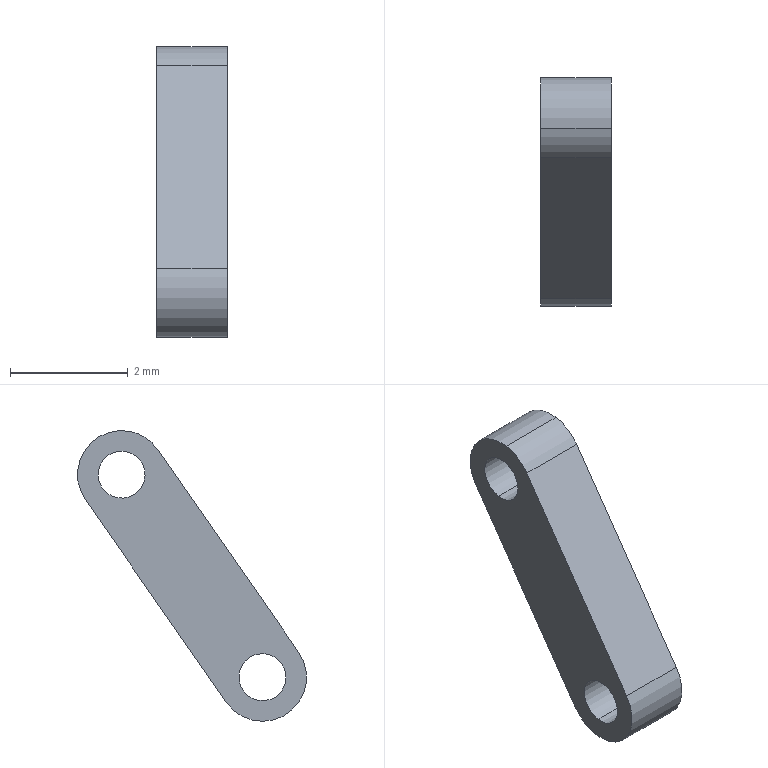Component | SolidWorks | RearWingYoke-4 | 1 solid | 11 faces | box 1.2 x 3.9 x 4.95 mm | volume 8 mm3 | cylinder 7 | plane 4 | commonest cylinder face diameters 0.8 x4 1.5 x3
build123d program:
from build123d import *

# Parameters (mm, degrees)
SKETCH1_R           = 0.4
BOSS_EXTRUDE1_DEPTH = 1.2


with BuildPart() as part:
    # Sketch1 → Boss-Extrude1 (new body)
    with BuildSketch(Plane.XY):
        with BuildLine():
            Line((-4.52, 1.96), (-7.547, 4.871))
            ThreePointArc((-7.547, 4.871), (-7.567, 5.932), (-6.507, 5.952))
            Line((-6.507, 5.952), (-3.48, 3.04))
            ThreePointArc((-3.48, 3.04), (-3.46, 1.98), (-4.52, 1.96))
        make_face()
        with Locations((-4, 2.5)):
            Circle(SKETCH1_R, mode=Mode.SUBTRACT)
        with Locations((-7.027, 5.412)):
            Circle(SKETCH1_R, mode=Mode.SUBTRACT)
    extrude(amount=BOSS_EXTRUDE1_DEPTH)


solid = part.part

# Placed as in the assembly
solid = solid.moved(Location((18.1, 10.831, 11.183), (-78.711, -90, 0)))
STEP:
#1=COLOUR_RGB('',0.7922,0.8196,0.9333);
#2=FILL_AREA_STYLE_COLOUR('',#1);
#3=FILL_AREA_STYLE('',(#2));
#4=SURFACE_STYLE_FILL_AREA(#3);
#5=SURFACE_SIDE_STYLE('',(#4));
#6=SURFACE_STYLE_USAGE(.BOTH.,#5);
#7=PRESENTATION_STYLE_ASSIGNMENT((#6));
#8=CARTESIAN_POINT('',(0.7126,0.2888,0.3285));
#9=VERTEX_POINT('',#8);
#10=CARTESIAN_POINT('',(0.7126,0.2938,0.2974));
#11=VERTEX_POINT('',#10);
#12=CARTESIAN_POINT('',(0.7126,0.2913,0.3129));
#13=DIRECTION('',(1.,0.,0.));
#14=DIRECTION('',(0.,0.1577,-0.9875));
#15=AXIS2_PLACEMENT_3D('',#12,#13,#14);
#16=CIRCLE('',#15,0.01575);
#17=EDGE_CURVE('',#9,#11,#16,.T.);
#18=ORIENTED_EDGE('',*,*,#17,.T.);
#19=CARTESIAN_POINT('',(0.6654,0.2938,0.2974));
#20=VERTEX_POINT('',#19);
#21=CARTESIAN_POINT('',(0.7126,0.2938,0.2974));
#22=DIRECTION('',(-1.,-0.,-0.));
#23=VECTOR('',#22,39.37);
#24=LINE('',#21,#23);
#25=EDGE_CURVE('',#11,#20,#24,.T.);
#26=ORIENTED_EDGE('',*,*,#25,.T.);
#27=CARTESIAN_POINT('',(0.6654,0.2888,0.3285));
#28=VERTEX_POINT('',#27);
#29=CARTESIAN_POINT('',(0.6654,0.2913,0.3129));
#30=DIRECTION('',(1.,0.,0.));
#31=DIRECTION('',(0.,0.1577,-0.9875));
#32=AXIS2_PLACEMENT_3D('',#29,#30,#31);
#33=CIRCLE('',#32,0.01575);
#34=EDGE_CURVE('',#28,#20,#33,.T.);
#35=ORIENTED_EDGE('',*,*,#34,.F.);
#36=CARTESIAN_POINT('',(0.7126,0.2888,0.3285));
#37=DIRECTION('',(-1.,-0.,-0.));
#38=VECTOR('',#37,39.37);
#39=LINE('',#36,#38);
#40=EDGE_CURVE('',#9,#28,#39,.T.);
#41=ORIENTED_EDGE('',*,*,#40,.F.);
#42=EDGE_LOOP('',(#18,#26,#35,#41));
#43=FACE_OUTER_BOUND('',#42,.T.);
#44=CARTESIAN_POINT('',(0.7126,0.2913,0.3129));
#45=DIRECTION('',(-1.,-0.,-0.));
#46=DIRECTION('',(0.,-0.1577,0.9875));
#47=AXIS2_PLACEMENT_3D('',#44,#45,#46);
#48=CYLINDRICAL_SURFACE('',#47,0.01575);
#49=ADVANCED_FACE('',(#43),#48,.F.);
#50=CARTESIAN_POINT('',(0.7126,0.1944,0.1927));
#51=VERTEX_POINT('',#50);
#52=CARTESIAN_POINT('',(0.7126,0.1993,0.1616));
#53=VERTEX_POINT('',#52);
#54=CARTESIAN_POINT('',(0.7126,0.1969,0.1772));
#55=DIRECTION('',(1.,0.,0.));
#56=DIRECTION('',(0.,0.1577,-0.9875));
#57=AXIS2_PLACEMENT_3D('',#54,#55,#56);
#58=CIRCLE('',#57,0.01575);
#59=EDGE_CURVE('',#51,#53,#58,.T.);
#60=ORIENTED_EDGE('',*,*,#59,.T.);
#61=CARTESIAN_POINT('',(0.6654,0.1993,0.1616));
#62=VERTEX_POINT('',#61);
#63=CARTESIAN_POINT('',(0.7126,0.1993,0.1616));
#64=DIRECTION('',(-1.,-0.,-0.));
#65=VECTOR('',#64,39.37);
#66=LINE('',#63,#65);
#67=EDGE_CURVE('',#53,#62,#66,.T.);
#68=ORIENTED_EDGE('',*,*,#67,.T.);
#69=CARTESIAN_POINT('',(0.6654,0.1944,0.1927));
#70=VERTEX_POINT('',#69);
#71=CARTESIAN_POINT('',(0.6654,0.1969,0.1772));
#72=DIRECTION('',(1.,0.,0.));
#73=DIRECTION('',(0.,0.1577,-0.9875));
#74=AXIS2_PLACEMENT_3D('',#71,#72,#73);
#75=CIRCLE('',#74,0.01575);
#76=EDGE_CURVE('',#70,#62,#75,.T.);
#77=ORIENTED_EDGE('',*,*,#76,.F.);
#78=CARTESIAN_POINT('',(0.7126,0.1944,0.1927));
#79=DIRECTION('',(-1.,-0.,-0.));
#80=VECTOR('',#79,39.37);
#81=LINE('',#78,#80);
#82=EDGE_CURVE('',#51,#70,#81,.T.);
#83=ORIENTED_EDGE('',*,*,#82,.F.);
#84=EDGE_LOOP('',(#60,#68,#77,#83));
#85=FACE_OUTER_BOUND('',#84,.T.);
#86=CARTESIAN_POINT('',(0.7126,0.1969,0.1772));
#87=DIRECTION('',(-1.,-0.,-0.));
#88=DIRECTION('',(0.,-0.1577,0.9875));
#89=AXIS2_PLACEMENT_3D('',#86,#87,#88);
#90=CYLINDRICAL_SURFACE('',#89,0.01575);
#91=ADVANCED_FACE('',(#85),#90,.F.);
#92=CARTESIAN_POINT('',(0.7126,0.2866,0.3421));
#93=VERTEX_POINT('',#92);
#94=CARTESIAN_POINT('',(0.7126,0.267,0.3298));
#95=VERTEX_POINT('',#94);
#96=CARTESIAN_POINT('',(0.7126,0.2913,0.3129));
#97=DIRECTION('',(1.,0.,0.));
#98=DIRECTION('',(0.,0.1577,-0.9875));
#99=AXIS2_PLACEMENT_3D('',#96,#97,#98);
#100=CIRCLE('',#99,0.02953);
#101=EDGE_CURVE('',#93,#95,#100,.T.);
#102=ORIENTED_EDGE('',*,*,#101,.F.);
#103=CARTESIAN_POINT('',(0.6654,0.2866,0.3421));
#104=VERTEX_POINT('',#103);
#105=CARTESIAN_POINT('',(0.7126,0.2866,0.3421));
#106=DIRECTION('',(-1.,-0.,-0.));
#107=VECTOR('',#106,39.37);
#108=LINE('',#105,#107);
#109=EDGE_CURVE('',#93,#104,#108,.T.);
#110=ORIENTED_EDGE('',*,*,#109,.T.);
#111=CARTESIAN_POINT('',(0.6654,0.267,0.3298));
#112=VERTEX_POINT('',#111);
#113=CARTESIAN_POINT('',(0.6654,0.2913,0.3129));
#114=DIRECTION('',(1.,0.,0.));
#115=DIRECTION('',(0.,0.1577,-0.9875));
#116=AXIS2_PLACEMENT_3D('',#113,#114,#115);
#117=CIRCLE('',#116,0.02953);
#118=EDGE_CURVE('',#104,#112,#117,.T.);
#119=ORIENTED_EDGE('',*,*,#118,.T.);
#120=CARTESIAN_POINT('',(0.7126,0.267,0.3298));
#121=DIRECTION('',(-1.,-0.,-0.));
#122=VECTOR('',#121,39.37);
#123=LINE('',#120,#122);
#124=EDGE_CURVE('',#95,#112,#123,.T.);
#125=ORIENTED_EDGE('',*,*,#124,.F.);
#126=EDGE_LOOP('',(#102,#110,#119,#125));
#127=FACE_OUTER_BOUND('',#126,.T.);
#128=CARTESIAN_POINT('',(0.7126,0.2913,0.3129));
#129=DIRECTION('',(-1.,-0.,-0.));
#130=DIRECTION('',(0.,-0.1577,0.9875));
#131=AXIS2_PLACEMENT_3D('',#128,#129,#130);
#132=CYLINDRICAL_SURFACE('',#131,0.02953);
#133=ADVANCED_FACE('',(#127),#132,.T.);
#134=ORIENTED_EDGE('',*,*,#59,.F.);
#135=CARTESIAN_POINT('',(0.7126,0.1969,0.1772));
#136=DIRECTION('',(1.,0.,0.));
#137=DIRECTION('',(0.,0.1577,-0.9875));
#138=AXIS2_PLACEMENT_3D('',#135,#136,#137);
#139=CIRCLE('',#138,0.01575);
#140=EDGE_CURVE('',#53,#51,#139,.T.);
#141=ORIENTED_EDGE('',*,*,#140,.F.);
#142=EDGE_LOOP('',(#134,#141));
#143=FACE_BOUND('',#142,.T.);
#144=CARTESIAN_POINT('',(0.7126,0.1726,0.194));
#145=VERTEX_POINT('',#144);
#146=CARTESIAN_POINT('',(0.7126,0.2211,0.1603));
#147=VERTEX_POINT('',#146);
#148=CARTESIAN_POINT('',(0.7126,0.1969,0.1772));
#149=DIRECTION('',(1.,0.,0.));
#150=DIRECTION('',(0.,0.1577,-0.9875));
#151=AXIS2_PLACEMENT_3D('',#148,#149,#150);
#152=CIRCLE('',#151,0.02953);
#153=EDGE_CURVE('',#145,#147,#152,.T.);
#154=ORIENTED_EDGE('',*,*,#153,.T.);
#155=CARTESIAN_POINT('',(0.7126,0.3155,0.2961));
#156=VERTEX_POINT('',#155);
#157=CARTESIAN_POINT('',(0.7126,0.2211,0.1603));
#158=DIRECTION('',(-0.,0.571,0.821));
#159=VECTOR('',#158,39.37);
#160=LINE('',#157,#159);
#161=EDGE_CURVE('',#147,#156,#160,.T.);
#162=ORIENTED_EDGE('',*,*,#161,.T.);
#163=CARTESIAN_POINT('',(0.7126,0.2913,0.3129));
#164=DIRECTION('',(1.,0.,0.));
#165=DIRECTION('',(0.,0.1577,-0.9875));
#166=AXIS2_PLACEMENT_3D('',#163,#164,#165);
#167=CIRCLE('',#166,0.02953);
#168=EDGE_CURVE('',#156,#93,#167,.T.);
#169=ORIENTED_EDGE('',*,*,#168,.T.);
#170=ORIENTED_EDGE('',*,*,#101,.T.);
#171=CARTESIAN_POINT('',(0.7126,0.1726,0.194));
#172=DIRECTION('',(0.,-0.571,-0.821));
#173=VECTOR('',#172,39.37);
#174=LINE('',#171,#173);
#175=EDGE_CURVE('',#95,#145,#174,.T.);
#176=ORIENTED_EDGE('',*,*,#175,.T.);
#177=EDGE_LOOP('',(#154,#162,#169,#170,#176));
#178=FACE_OUTER_BOUND('',#177,.T.);
#179=ORIENTED_EDGE('',*,*,#17,.F.);
#180=CARTESIAN_POINT('',(0.7126,0.2913,0.3129));
#181=DIRECTION('',(1.,0.,0.));
#182=DIRECTION('',(0.,0.1577,-0.9875));
#183=AXIS2_PLACEMENT_3D('',#180,#181,#182);
#184=CIRCLE('',#183,0.01575);
#185=EDGE_CURVE('',#11,#9,#184,.T.);
#186=ORIENTED_EDGE('',*,*,#185,.F.);
#187=EDGE_LOOP('',(#179,#186));
#188=FACE_BOUND('',#187,.T.);
#189=CARTESIAN_POINT('',(0.7126,0.1969,0.1772));
#190=DIRECTION('',(1.,0.,0.));
#191=DIRECTION('',(0.,0.1577,-0.9875));
#192=AXIS2_PLACEMENT_3D('',#189,#190,#191);
#193=PLANE('',#192);
#194=ADVANCED_FACE('',(#143,#178,#188),#193,.T.);
#195=CARTESIAN_POINT('',(0.6654,0.1726,0.194));
#196=VERTEX_POINT('',#195);
#197=CARTESIAN_POINT('',(0.6654,0.2211,0.1603));
#198=VERTEX_POINT('',#197);
#199=CARTESIAN_POINT('',(0.6654,0.1969,0.1772));
#200=DIRECTION('',(1.,0.,0.));
#201=DIRECTION('',(0.,0.1577,-0.9875));
#202=AXIS2_PLACEMENT_3D('',#199,#200,#201);
#203=CIRCLE('',#202,0.02953);
#204=EDGE_CURVE('',#196,#198,#203,.T.);
#205=ORIENTED_EDGE('',*,*,#204,.F.);
#206=CARTESIAN_POINT('',(0.6654,0.1726,0.194));
#207=DIRECTION('',(0.,-0.571,-0.821));
#208=VECTOR('',#207,39.37);
#209=LINE('',#206,#208);
#210=EDGE_CURVE('',#112,#196,#209,.T.);
#211=ORIENTED_EDGE('',*,*,#210,.F.);
#212=ORIENTED_EDGE('',*,*,#118,.F.);
#213=CARTESIAN_POINT('',(0.6654,0.3155,0.2961));
#214=VERTEX_POINT('',#213);
#215=CARTESIAN_POINT('',(0.6654,0.2913,0.3129));
#216=DIRECTION('',(1.,0.,0.));
#217=DIRECTION('',(0.,0.1577,-0.9875));
#218=AXIS2_PLACEMENT_3D('',#215,#216,#217);
#219=CIRCLE('',#218,0.02953);
#220=EDGE_CURVE('',#214,#104,#219,.T.);
#221=ORIENTED_EDGE('',*,*,#220,.F.);
#222=CARTESIAN_POINT('',(0.6654,0.2211,0.1603));
#223=DIRECTION('',(-0.,0.571,0.821));
#224=VECTOR('',#223,39.37);
#225=LINE('',#222,#224);
#226=EDGE_CURVE('',#198,#214,#225,.T.);
#227=ORIENTED_EDGE('',*,*,#226,.F.);
#228=EDGE_LOOP('',(#205,#211,#212,#221,#227));
#229=FACE_OUTER_BOUND('',#228,.T.);
#230=ORIENTED_EDGE('',*,*,#76,.T.);
#231=CARTESIAN_POINT('',(0.6654,0.1969,0.1772));
#232=DIRECTION('',(1.,0.,0.));
#233=DIRECTION('',(0.,0.1577,-0.9875));
#234=AXIS2_PLACEMENT_3D('',#231,#232,#233);
#235=CIRCLE('',#234,0.01575);
#236=EDGE_CURVE('',#62,#70,#235,.T.);
#237=ORIENTED_EDGE('',*,*,#236,.T.);
#238=EDGE_LOOP('',(#230,#237));
#239=FACE_BOUND('',#238,.T.);
#240=ORIENTED_EDGE('',*,*,#34,.T.);
#241=CARTESIAN_POINT('',(0.6654,0.2913,0.3129));
#242=DIRECTION('',(1.,0.,0.));
#243=DIRECTION('',(0.,0.1577,-0.9875));
#244=AXIS2_PLACEMENT_3D('',#241,#242,#243);
#245=CIRCLE('',#244,0.01575);
#246=EDGE_CURVE('',#20,#28,#245,.T.);
#247=ORIENTED_EDGE('',*,*,#246,.T.);
#248=EDGE_LOOP('',(#240,#247));
#249=FACE_BOUND('',#248,.T.);
#250=CARTESIAN_POINT('',(0.6654,0.1969,0.1772));
#251=DIRECTION('',(1.,0.,0.));
#252=DIRECTION('',(0.,0.1577,-0.9875));
#253=AXIS2_PLACEMENT_3D('',#250,#251,#252);
#254=PLANE('',#253);
#255=ADVANCED_FACE('',(#229,#239,#249),#254,.F.);
#256=ORIENTED_EDGE('',*,*,#204,.T.);
#257=CARTESIAN_POINT('',(0.7126,0.2211,0.1603));
#258=DIRECTION('',(-1.,-0.,-0.));
#259=VECTOR('',#258,39.37);
#260=LINE('',#257,#259);
#261=EDGE_CURVE('',#147,#198,#260,.T.);
#262=ORIENTED_EDGE('',*,*,#261,.F.);
#263=ORIENTED_EDGE('',*,*,#153,.F.);
#264=CARTESIAN_POINT('',(0.7126,0.1726,0.194));
#265=DIRECTION('',(-1.,-0.,-0.));
#266=VECTOR('',#265,39.37);
#267=LINE('',#264,#266);
#268=EDGE_CURVE('',#145,#196,#267,.T.);
#269=ORIENTED_EDGE('',*,*,#268,.T.);
#270=EDGE_LOOP('',(#256,#262,#263,#269));
#271=FACE_OUTER_BOUND('',#270,.T.);
#272=CARTESIAN_POINT('',(0.7126,0.1969,0.1772));
#273=DIRECTION('',(-1.,-0.,-0.));
#274=DIRECTION('',(0.,-0.1577,0.9875));
#275=AXIS2_PLACEMENT_3D('',#272,#273,#274);
#276=CYLINDRICAL_SURFACE('',#275,0.02953);
#277=ADVANCED_FACE('',(#271),#276,.T.);
#278=ORIENTED_EDGE('',*,*,#226,.T.);
#279=CARTESIAN_POINT('',(0.7126,0.3155,0.2961));
#280=DIRECTION('',(-1.,-0.,-0.));
#281=VECTOR('',#280,39.37);
#282=LINE('',#279,#281);
#283=EDGE_CURVE('',#156,#214,#282,.T.);
#284=ORIENTED_EDGE('',*,*,#283,.F.);
#285=ORIENTED_EDGE('',*,*,#161,.F.);
#286=ORIENTED_EDGE('',*,*,#261,.T.);
#287=EDGE_LOOP('',(#278,#284,#285,#286));
#288=FACE_OUTER_BOUND('',#287,.T.);
#289=CARTESIAN_POINT('',(0.7126,0.2211,0.1603));
#290=DIRECTION('',(0.,-0.821,0.571));
#291=DIRECTION('',(0.,-0.571,-0.821));
#292=AXIS2_PLACEMENT_3D('',#289,#290,#291);
#293=PLANE('',#292);
#294=ADVANCED_FACE('',(#288),#293,.F.);
#295=ORIENTED_EDGE('',*,*,#109,.F.);
#296=ORIENTED_EDGE('',*,*,#168,.F.);
#297=ORIENTED_EDGE('',*,*,#283,.T.);
#298=ORIENTED_EDGE('',*,*,#220,.T.);
#299=EDGE_LOOP('',(#295,#296,#297,#298));
#300=FACE_OUTER_BOUND('',#299,.T.);
#301=CARTESIAN_POINT('',(0.7126,0.2913,0.3129));
#302=DIRECTION('',(-1.,-0.,-0.));
#303=DIRECTION('',(0.,-0.1577,0.9875));
#304=AXIS2_PLACEMENT_3D('',#301,#302,#303);
#305=CYLINDRICAL_SURFACE('',#304,0.02953);
#306=ADVANCED_FACE('',(#300),#305,.T.);
#307=ORIENTED_EDGE('',*,*,#210,.T.);
#308=ORIENTED_EDGE('',*,*,#268,.F.);
#309=ORIENTED_EDGE('',*,*,#175,.F.);
#310=ORIENTED_EDGE('',*,*,#124,.T.);
#311=EDGE_LOOP('',(#307,#308,#309,#310));
#312=FACE_OUTER_BOUND('',#311,.T.);
#313=CARTESIAN_POINT('',(0.7126,0.1726,0.194));
#314=DIRECTION('',(-0.,0.821,-0.571));
#315=DIRECTION('',(-0.,0.571,0.821));
#316=AXIS2_PLACEMENT_3D('',#313,#314,#315);
#317=PLANE('',#316);
#318=ADVANCED_FACE('',(#312),#317,.F.);
#319=ORIENTED_EDGE('',*,*,#67,.F.);
#320=ORIENTED_EDGE('',*,*,#140,.T.);
#321=ORIENTED_EDGE('',*,*,#82,.T.);
#322=ORIENTED_EDGE('',*,*,#236,.F.);
#323=EDGE_LOOP('',(#319,#320,#321,#322));
#324=FACE_OUTER_BOUND('',#323,.T.);
#325=CARTESIAN_POINT('',(0.7126,0.1969,0.1772));
#326=DIRECTION('',(-1.,-0.,-0.));
#327=DIRECTION('',(0.,-0.1577,0.9875));
#328=AXIS2_PLACEMENT_3D('',#325,#326,#327);
#329=CYLINDRICAL_SURFACE('',#328,0.01575);
#330=ADVANCED_FACE('',(#324),#329,.F.);
#331=ORIENTED_EDGE('',*,*,#25,.F.);
#332=ORIENTED_EDGE('',*,*,#185,.T.);
#333=ORIENTED_EDGE('',*,*,#40,.T.);
#334=ORIENTED_EDGE('',*,*,#246,.F.);
#335=EDGE_LOOP('',(#331,#332,#333,#334));
#336=FACE_OUTER_BOUND('',#335,.T.);
#337=CARTESIAN_POINT('',(0.7126,0.2913,0.3129));
#338=DIRECTION('',(-1.,-0.,-0.));
#339=DIRECTION('',(0.,-0.1577,0.9875));
#340=AXIS2_PLACEMENT_3D('',#337,#338,#339);
#341=CYLINDRICAL_SURFACE('',#340,0.01575);
#342=ADVANCED_FACE('',(#336),#341,.F.);
#343=CLOSED_SHELL('',(#49,#91,#133,#194,#255,#277,#294,#306,#318,#330,#342));
#344=MANIFOLD_SOLID_BREP('',#343);
#345=STYLED_ITEM('',(#7),#344);
#346=PRESENTATION_LAYER_ASSIGNMENT('','',(#345));
#347=CARTESIAN_POINT('',(0.,0.,0.));
#348=DIRECTION('',(0.,0.,1.));
#349=DIRECTION('',(1.,0.,0.));
#350=AXIS2_PLACEMENT_3D('',#347,#348,#349);
#351=(LENGTH_UNIT()NAMED_UNIT(*)SI_UNIT($,.METRE.));
#352=LENGTH_MEASURE_WITH_UNIT(LENGTH_MEASURE(0.0254),#351);
#353=DIMENSIONAL_EXPONENTS(1.,0.,0.,0.,0.,0.,0.);
#354=(CONVERSION_BASED_UNIT('',#352)LENGTH_UNIT()NAMED_UNIT(#353));
#355=UNCERTAINTY_MEASURE_WITH_UNIT(LENGTH_MEASURE(0.00001),#354,'','');
#356=(NAMED_UNIT(*)PLANE_ANGLE_UNIT()SI_UNIT($,.RADIAN.));
#357=(NAMED_UNIT(*)SI_UNIT($,.STERADIAN.)SOLID_ANGLE_UNIT());
#358=(GEOMETRIC_REPRESENTATION_CONTEXT(3)GLOBAL_UNCERTAINTY_ASSIGNED_CONTEXT((#355))GLOBAL_UNIT_ASSIGNED_CONTEXT((#354,#356,#357))REPRESENTATION_CONTEXT('',''));
#359=ADVANCED_BREP_SHAPE_REPRESENTATION('',(#344,#350),#358);
#360=(LENGTH_UNIT()NAMED_UNIT(*)SI_UNIT($,.METRE.));
#361=LENGTH_MEASURE_WITH_UNIT(LENGTH_MEASURE(0.0254),#360);
#362=DIMENSIONAL_EXPONENTS(1.,0.,0.,0.,0.,0.,0.);
#363=(CONVERSION_BASED_UNIT('',#361)LENGTH_UNIT()NAMED_UNIT(#362));
#364=UNCERTAINTY_MEASURE_WITH_UNIT(LENGTH_MEASURE(0.00001),#363,'','');
#365=(NAMED_UNIT(*)PLANE_ANGLE_UNIT()SI_UNIT($,.RADIAN.));
#366=(NAMED_UNIT(*)SI_UNIT($,.STERADIAN.)SOLID_ANGLE_UNIT());
#367=(GEOMETRIC_REPRESENTATION_CONTEXT(3)GLOBAL_UNCERTAINTY_ASSIGNED_CONTEXT((#364))GLOBAL_UNIT_ASSIGNED_CONTEXT((#363,#365,#366))REPRESENTATION_CONTEXT('',''));
#368=MECHANICAL_DESIGN_GEOMETRIC_PRESENTATION_REPRESENTATION('',(#345),#367);